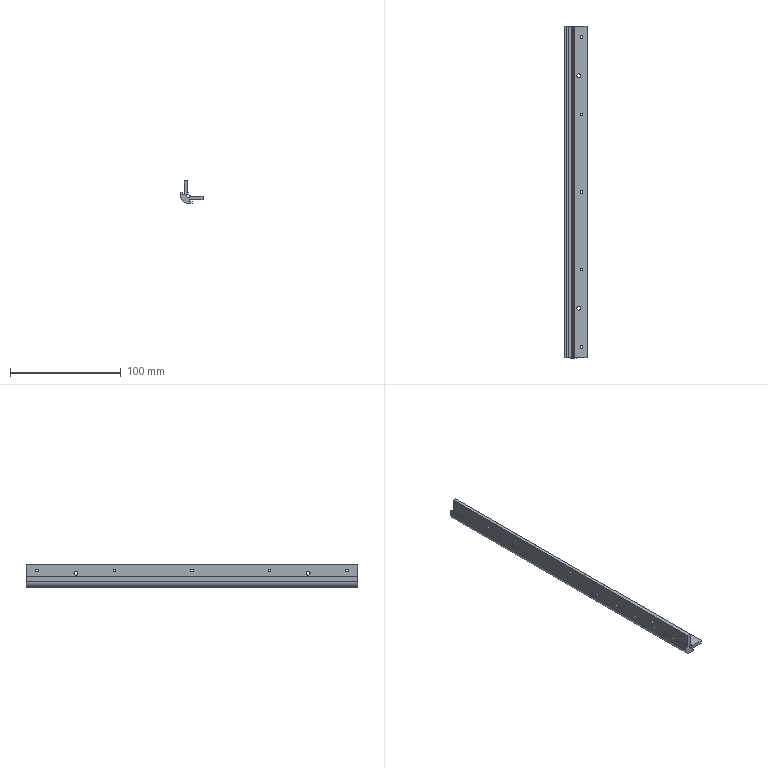CAM job | Mastercam | mm | 6 operations | part box 20 x 300 x 20
1. Contour (Ramp) | 6 - 6 平铣刀
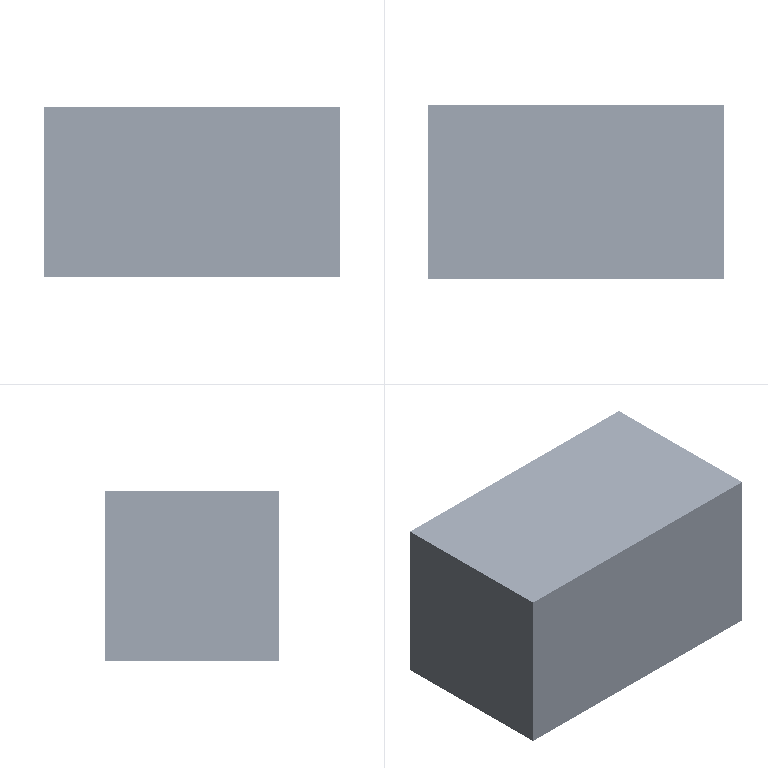2. Contour (2D) | 6 - 6 平铣刀
3. Drill/Counterbore | 5 - 4 倒角刀
4. Contour (Ramp) | 6 - 6 平铣刀
5. Contour (2D) | 6 - 6 平铣刀
6. Drill/Counterbore | 5 - 4 倒角刀